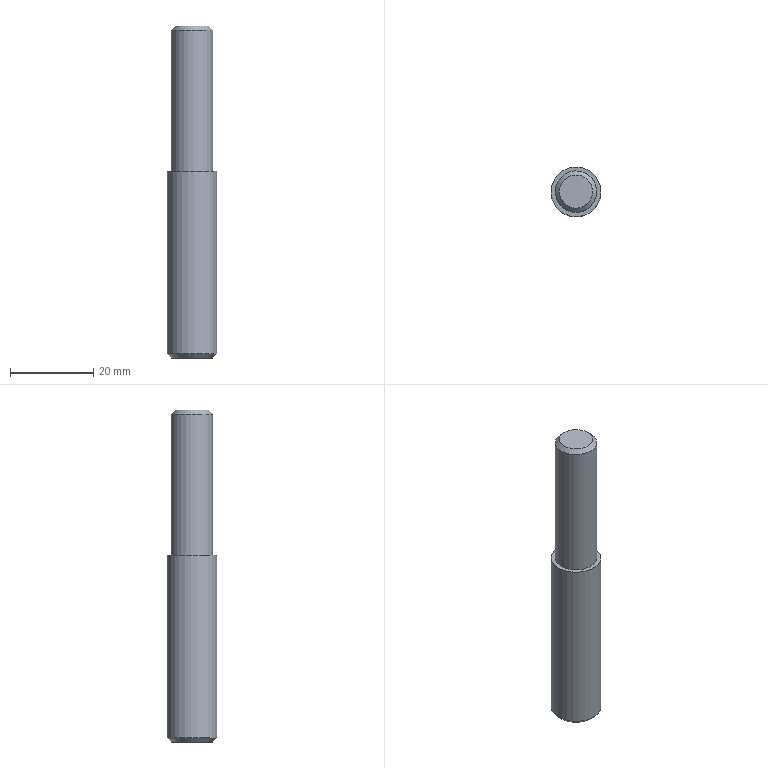Component | NX | PIN_FOR_TOGGLE_LEVER_2 | 1 solid | 7 faces | box 12 x 12 x 80 mm | volume 7806 mm3 | plane 3 | cylinder 2 | cone 2 | commonest cylinder face diameters 12 x1 10 x1
STEP:
#1=CARTESIAN_POINT('',(0.,0.,0.));
#2=DIRECTION('',(0.,0.,1.));
#3=DIRECTION('',(1.,0.,0.));
#4=AXIS2_PLACEMENT_3D('',#1,#2,#3);
#5=CARTESIAN_POINT('',(-2.434,171.826,43.728));
#6=VERTEX_POINT('',#5);
#7=CARTESIAN_POINT('',(0.,175.,43.728));
#8=DIRECTION('',(0.,0.,1.));
#9=DIRECTION('',(-0.6084,-0.7936,0.));
#10=AXIS2_PLACEMENT_3D('',#7,#8,#9);
#11=CIRCLE('',#10,4.);
#12=CARTESIAN_POINT('',(3.968,171.958,43.728));
#13=DIRECTION('',(0.,0.,1.));
#14=DIRECTION('',(-0.6084,-0.7936,0.));
#15=AXIS2_PLACEMENT_3D('',#12,#13,#14);
#16=PLANE('',#15);
#17=CARTESIAN_POINT('',(-0.,-5.));
#18=DIRECTION('',(1.,-0.));
#19=AXIS2_PLACEMENT_2D('',#17,#18);
#20=CIRCLE('',#19,4.);
#21=(GEOMETRIC_REPRESENTATION_CONTEXT(2)PARAMETRIC_REPRESENTATION_CONTEXT()REPRESENTATION_CONTEXT('',''));
#22=DEFINITIONAL_REPRESENTATION('',(#20),#21);
#23=PCURVE('',#16,#22);
#24=CARTESIAN_POINT('',(0.,175.,42.728));
#25=DIRECTION('',(0.,0.,-1.));
#26=DIRECTION('',(0.6084,0.7936,0.));
#27=AXIS2_PLACEMENT_3D('',#24,#25,#26);
#28=CONICAL_SURFACE('',#27,5.,0.7854);
#29=CARTESIAN_POINT('',(9.425,-1.));
#30=DIRECTION('',(-1.,0.));
#31=VECTOR('',#30,1.);
#32=LINE('',#29,#31);
#33=(GEOMETRIC_REPRESENTATION_CONTEXT(2)PARAMETRIC_REPRESENTATION_CONTEXT()REPRESENTATION_CONTEXT('',''));
#34=DEFINITIONAL_REPRESENTATION('',(#32),#33);
#35=PCURVE('',#28,#34);
#36=SURFACE_CURVE('',#11,(#23,#35),.PCURVE_S1.);
#37=EDGE_CURVE('',#6,#6,#36,.T.);
#38=ORIENTED_EDGE('',*,*,#37,.T.);
#39=EDGE_LOOP('',(#38));
#40=FACE_BOUND('',#39,.T.);
#41=ADVANCED_FACE('',(#40),#16,.T.);
#42=CARTESIAN_POINT('',(3.042,178.968,-36.272));
#43=VERTEX_POINT('',#42);
#44=CARTESIAN_POINT('',(0.,175.,-36.272));
#45=DIRECTION('',(0.,0.,-1.));
#46=DIRECTION('',(0.6084,0.7936,0.));
#47=AXIS2_PLACEMENT_3D('',#44,#45,#46);
#48=CIRCLE('',#47,5.);
#49=CARTESIAN_POINT('',(0.,175.,-36.272));
#50=DIRECTION('',(0.,0.,-1.));
#51=DIRECTION('',(0.6084,0.7936,0.));
#52=AXIS2_PLACEMENT_3D('',#49,#50,#51);
#53=PLANE('',#52);
#54=CARTESIAN_POINT('',(0.,0.));
#55=DIRECTION('',(1.,-0.));
#56=AXIS2_PLACEMENT_2D('',#54,#55);
#57=CIRCLE('',#56,5.);
#58=(GEOMETRIC_REPRESENTATION_CONTEXT(2)PARAMETRIC_REPRESENTATION_CONTEXT()REPRESENTATION_CONTEXT('',''));
#59=DEFINITIONAL_REPRESENTATION('',(#57),#58);
#60=PCURVE('',#53,#59);
#61=CARTESIAN_POINT('',(0.,175.,-36.272));
#62=DIRECTION('',(0.,0.,1.));
#63=DIRECTION('',(-0.6084,-0.7936,0.));
#64=AXIS2_PLACEMENT_3D('',#61,#62,#63);
#65=CONICAL_SURFACE('',#64,5.,0.7854);
#66=CARTESIAN_POINT('',(9.425,-0.));
#67=DIRECTION('',(-1.,0.));
#68=VECTOR('',#67,1.);
#69=LINE('',#66,#68);
#70=(GEOMETRIC_REPRESENTATION_CONTEXT(2)PARAMETRIC_REPRESENTATION_CONTEXT()REPRESENTATION_CONTEXT('',''));
#71=DEFINITIONAL_REPRESENTATION('',(#69),#70);
#72=PCURVE('',#65,#71);
#73=SURFACE_CURVE('',#48,(#60,#72),.PCURVE_S1.);
#74=EDGE_CURVE('',#43,#43,#73,.T.);
#75=ORIENTED_EDGE('',*,*,#74,.T.);
#76=EDGE_LOOP('',(#75));
#77=FACE_BOUND('',#76,.T.);
#78=ADVANCED_FACE('',(#77),#53,.T.);
#79=CARTESIAN_POINT('',(3.651,179.762,-35.272));
#80=VERTEX_POINT('',#79);
#81=CARTESIAN_POINT('',(0.,175.,-35.272));
#82=DIRECTION('',(0.,0.,1.));
#83=DIRECTION('',(0.6084,0.7936,0.));
#84=AXIS2_PLACEMENT_3D('',#81,#82,#83);
#85=CIRCLE('',#84,6.);
#86=CARTESIAN_POINT('',(0.,175.,-36.272));
#87=DIRECTION('',(0.,0.,-1.));
#88=DIRECTION('',(0.6084,0.7936,0.));
#89=AXIS2_PLACEMENT_3D('',#86,#87,#88);
#90=CYLINDRICAL_SURFACE('',#89,6.);
#91=CARTESIAN_POINT('',(6.283,-1.));
#92=DIRECTION('',(-1.,0.));
#93=VECTOR('',#92,1.);
#94=LINE('',#91,#93);
#95=(GEOMETRIC_REPRESENTATION_CONTEXT(2)PARAMETRIC_REPRESENTATION_CONTEXT()REPRESENTATION_CONTEXT('',''));
#96=DEFINITIONAL_REPRESENTATION('',(#94),#95);
#97=PCURVE('',#90,#96);
#98=CARTESIAN_POINT('',(3.142,1.));
#99=DIRECTION('',(1.,0.));
#100=VECTOR('',#99,1.);
#101=LINE('',#98,#100);
#102=(GEOMETRIC_REPRESENTATION_CONTEXT(2)PARAMETRIC_REPRESENTATION_CONTEXT()REPRESENTATION_CONTEXT('',''));
#103=DEFINITIONAL_REPRESENTATION('',(#101),#102);
#104=PCURVE('',#65,#103);
#105=SURFACE_CURVE('',#85,(#97,#104),.PCURVE_S1.);
#106=EDGE_CURVE('',#80,#80,#105,.T.);
#107=ORIENTED_EDGE('',*,*,#106,.T.);
#108=CARTESIAN_POINT('',(3.651,179.762,8.728));
#109=VERTEX_POINT('',#108);
#110=CARTESIAN_POINT('',(3.651,179.762,8.728));
#111=CARTESIAN_POINT('',(3.651,179.762,-35.272));
#112=B_SPLINE_CURVE_WITH_KNOTS('',1,(#110,#111),.UNSPECIFIED.,.F.,.F.,(2,2),(-45.,-1.),.PIECEWISE_BEZIER_KNOTS.);
#113=CARTESIAN_POINT('',(0.,0.));
#114=DIRECTION('',(0.,1.));
#115=VECTOR('',#114,1.);
#116=LINE('',#113,#115);
#117=(GEOMETRIC_REPRESENTATION_CONTEXT(2)PARAMETRIC_REPRESENTATION_CONTEXT()REPRESENTATION_CONTEXT('',''));
#118=DEFINITIONAL_REPRESENTATION('',(#116),#117);
#119=PCURVE('',#90,#118);
#120=CARTESIAN_POINT('',(6.283,0.));
#121=DIRECTION('',(0.,1.));
#122=VECTOR('',#121,1.);
#123=LINE('',#120,#122);
#124=(GEOMETRIC_REPRESENTATION_CONTEXT(2)PARAMETRIC_REPRESENTATION_CONTEXT()REPRESENTATION_CONTEXT('',''));
#125=DEFINITIONAL_REPRESENTATION('',(#123),#124);
#126=PCURVE('',#90,#125);
#127=SEAM_CURVE('',#112,(#119,#126),.PCURVE_S1.);
#128=EDGE_CURVE('',#109,#80,#127,.T.);
#129=ORIENTED_EDGE('',*,*,#128,.F.);
#130=CARTESIAN_POINT('',(0.,175.,8.728));
#131=DIRECTION('',(0.,0.,-1.));
#132=DIRECTION('',(0.6084,0.7936,0.));
#133=AXIS2_PLACEMENT_3D('',#130,#131,#132);
#134=CIRCLE('',#133,6.);
#135=CARTESIAN_POINT('',(0.,-45.));
#136=DIRECTION('',(1.,0.));
#137=VECTOR('',#136,1.);
#138=LINE('',#135,#137);
#139=(GEOMETRIC_REPRESENTATION_CONTEXT(2)PARAMETRIC_REPRESENTATION_CONTEXT()REPRESENTATION_CONTEXT('',''));
#140=DEFINITIONAL_REPRESENTATION('',(#138),#139);
#141=PCURVE('',#90,#140);
#142=CARTESIAN_POINT('',(4.762,171.349,8.728));
#143=DIRECTION('',(0.,0.,1.));
#144=DIRECTION('',(-0.6084,-0.7936,0.));
#145=AXIS2_PLACEMENT_3D('',#142,#143,#144);
#146=PLANE('',#145);
#147=CARTESIAN_POINT('',(-6.,-6.));
#148=CARTESIAN_POINT('',(-6.,4.392));
#149=CARTESIAN_POINT('',(3.,-0.8038));
#150=CARTESIAN_POINT('',(12.,-6.));
#151=CARTESIAN_POINT('',(3.,-11.196));
#152=CARTESIAN_POINT('',(-6.,-16.392));
#153=CARTESIAN_POINT('',(-6.,-6.));
#154=(BOUNDED_CURVE()B_SPLINE_CURVE(2,(#147,#148,#149,#150,#151,#152,#153),.UNSPECIFIED.,.T.,.F.)B_SPLINE_CURVE_WITH_KNOTS((1,2,2,2,2,1),(-2.094,0.,2.094,4.189,6.283,8.378),.UNSPECIFIED.)CURVE()GEOMETRIC_REPRESENTATION_ITEM()RATIONAL_B_SPLINE_CURVE((1.,0.5,1.,0.5,1.,0.5,1.))REPRESENTATION_ITEM(''));
#155=(GEOMETRIC_REPRESENTATION_CONTEXT(2)PARAMETRIC_REPRESENTATION_CONTEXT()REPRESENTATION_CONTEXT('',''));
#156=DEFINITIONAL_REPRESENTATION('',(#154),#155);
#157=PCURVE('',#146,#156);
#158=SURFACE_CURVE('',#134,(#141,#157),.PCURVE_S1.);
#159=EDGE_CURVE('',#109,#109,#158,.T.);
#160=ORIENTED_EDGE('',*,*,#159,.T.);
#161=ORIENTED_EDGE('',*,*,#128,.T.);
#162=EDGE_LOOP('',(#107,#129,#160,#161));
#163=FACE_BOUND('',#162,.T.);
#164=ADVANCED_FACE('',(#163),#90,.T.);
#165=CARTESIAN_POINT('',(3.042,178.968,8.728));
#166=VERTEX_POINT('',#165);
#167=CARTESIAN_POINT('',(0.,175.,8.728));
#168=DIRECTION('',(0.,0.,-1.));
#169=DIRECTION('',(0.6084,0.7936,0.));
#170=AXIS2_PLACEMENT_3D('',#167,#168,#169);
#171=CIRCLE('',#170,5.);
#172=CARTESIAN_POINT('',(-5.,-6.));
#173=CARTESIAN_POINT('',(-5.,2.66));
#174=CARTESIAN_POINT('',(2.5,-1.67));
#175=CARTESIAN_POINT('',(10.,-6.));
#176=CARTESIAN_POINT('',(2.5,-10.33));
#177=CARTESIAN_POINT('',(-5.,-14.66));
#178=CARTESIAN_POINT('',(-5.,-6.));
#179=(BOUNDED_CURVE()B_SPLINE_CURVE(2,(#172,#173,#174,#175,#176,#177,#178),.UNSPECIFIED.,.T.,.F.)B_SPLINE_CURVE_WITH_KNOTS((1,2,2,2,2,1),(-2.094,0.,2.094,4.189,6.283,8.378),.UNSPECIFIED.)CURVE()GEOMETRIC_REPRESENTATION_ITEM()RATIONAL_B_SPLINE_CURVE((1.,0.5,1.,0.5,1.,0.5,1.))REPRESENTATION_ITEM(''));
#180=(GEOMETRIC_REPRESENTATION_CONTEXT(2)PARAMETRIC_REPRESENTATION_CONTEXT()REPRESENTATION_CONTEXT('',''));
#181=DEFINITIONAL_REPRESENTATION('',(#179),#180);
#182=PCURVE('',#146,#181);
#183=CARTESIAN_POINT('',(0.,175.,-36.272));
#184=DIRECTION('',(0.,0.,-1.));
#185=DIRECTION('',(0.6084,0.7936,0.));
#186=AXIS2_PLACEMENT_3D('',#183,#184,#185);
#187=CYLINDRICAL_SURFACE('',#186,5.);
#188=CARTESIAN_POINT('',(0.,-45.));
#189=DIRECTION('',(1.,0.));
#190=VECTOR('',#189,1.);
#191=LINE('',#188,#190);
#192=(GEOMETRIC_REPRESENTATION_CONTEXT(2)PARAMETRIC_REPRESENTATION_CONTEXT()REPRESENTATION_CONTEXT('',''));
#193=DEFINITIONAL_REPRESENTATION('',(#191),#192);
#194=PCURVE('',#187,#193);
#195=SURFACE_CURVE('',#171,(#182,#194),.PCURVE_S1.);
#196=EDGE_CURVE('',#166,#166,#195,.T.);
#197=ORIENTED_EDGE('',*,*,#196,.T.);
#198=EDGE_LOOP('',(#197));
#199=FACE_BOUND('',#198,.T.);
#200=ORIENTED_EDGE('',*,*,#159,.F.);
#201=EDGE_LOOP('',(#200));
#202=FACE_BOUND('',#201,.T.);
#203=ADVANCED_FACE('',(#199,#202),#146,.T.);
#204=CARTESIAN_POINT('',(-3.042,171.032,42.728));
#205=VERTEX_POINT('',#204);
#206=CARTESIAN_POINT('',(3.042,178.968,42.728));
#207=VERTEX_POINT('',#206);
#208=CARTESIAN_POINT('',(0.,175.,42.728));
#209=DIRECTION('',(0.,0.,-1.));
#210=DIRECTION('',(-0.6084,-0.7936,0.));
#211=AXIS2_PLACEMENT_3D('',#208,#209,#210);
#212=CIRCLE('',#211,5.);
#213=CARTESIAN_POINT('',(3.142,-79.));
#214=DIRECTION('',(1.,0.));
#215=VECTOR('',#214,1.);
#216=LINE('',#213,#215);
#217=(GEOMETRIC_REPRESENTATION_CONTEXT(2)PARAMETRIC_REPRESENTATION_CONTEXT()REPRESENTATION_CONTEXT('',''));
#218=DEFINITIONAL_REPRESENTATION('',(#216),#217);
#219=PCURVE('',#187,#218);
#220=CARTESIAN_POINT('',(3.142,0.));
#221=DIRECTION('',(1.,-0.));
#222=VECTOR('',#221,1.);
#223=LINE('',#220,#222);
#224=(GEOMETRIC_REPRESENTATION_CONTEXT(2)PARAMETRIC_REPRESENTATION_CONTEXT()REPRESENTATION_CONTEXT('',''));
#225=DEFINITIONAL_REPRESENTATION('',(#223),#224);
#226=PCURVE('',#28,#225);
#227=SURFACE_CURVE('',#212,(#219,#226),.PCURVE_S1.);
#228=EDGE_CURVE('',#205,#207,#227,.T.);
#229=ORIENTED_EDGE('',*,*,#228,.T.);
#230=CARTESIAN_POINT('',(3.042,178.968,42.728));
#231=CARTESIAN_POINT('',(3.042,178.968,8.728));
#232=B_SPLINE_CURVE_WITH_KNOTS('',1,(#230,#231),.UNSPECIFIED.,.F.,.F.,(2,2),(-79.,-45.),.PIECEWISE_BEZIER_KNOTS.);
#233=CARTESIAN_POINT('',(6.283,0.));
#234=DIRECTION('',(0.,1.));
#235=VECTOR('',#234,1.);
#236=LINE('',#233,#235);
#237=(GEOMETRIC_REPRESENTATION_CONTEXT(2)PARAMETRIC_REPRESENTATION_CONTEXT()REPRESENTATION_CONTEXT('',''));
#238=DEFINITIONAL_REPRESENTATION('',(#236),#237);
#239=PCURVE('',#187,#238);
#240=CARTESIAN_POINT('',(0.,0.));
#241=DIRECTION('',(0.,1.));
#242=VECTOR('',#241,1.);
#243=LINE('',#240,#242);
#244=(GEOMETRIC_REPRESENTATION_CONTEXT(2)PARAMETRIC_REPRESENTATION_CONTEXT()REPRESENTATION_CONTEXT('',''));
#245=DEFINITIONAL_REPRESENTATION('',(#243),#244);
#246=PCURVE('',#187,#245);
#247=SEAM_CURVE('',#232,(#239,#246),.PCURVE_S1.);
#248=EDGE_CURVE('',#207,#166,#247,.T.);
#249=ORIENTED_EDGE('',*,*,#248,.T.);
#250=ORIENTED_EDGE('',*,*,#196,.F.);
#251=ORIENTED_EDGE('',*,*,#248,.F.);
#252=CARTESIAN_POINT('',(0.,175.,42.728));
#253=DIRECTION('',(0.,0.,-1.));
#254=DIRECTION('',(-0.6084,-0.7936,0.));
#255=AXIS2_PLACEMENT_3D('',#252,#253,#254);
#256=CIRCLE('',#255,5.);
#257=CARTESIAN_POINT('',(-3.142,-79.));
#258=DIRECTION('',(1.,0.));
#259=VECTOR('',#258,1.);
#260=LINE('',#257,#259);
#261=(GEOMETRIC_REPRESENTATION_CONTEXT(2)PARAMETRIC_REPRESENTATION_CONTEXT()REPRESENTATION_CONTEXT('',''));
#262=DEFINITIONAL_REPRESENTATION('',(#260),#261);
#263=PCURVE('',#187,#262);
#264=CARTESIAN_POINT('',(3.142,-0.));
#265=DIRECTION('',(1.,0.));
#266=VECTOR('',#265,1.);
#267=LINE('',#264,#266);
#268=(GEOMETRIC_REPRESENTATION_CONTEXT(2)PARAMETRIC_REPRESENTATION_CONTEXT()REPRESENTATION_CONTEXT('',''));
#269=DEFINITIONAL_REPRESENTATION('',(#267),#268);
#270=PCURVE('',#28,#269);
#271=SURFACE_CURVE('',#256,(#263,#270),.PCURVE_S1.);
#272=EDGE_CURVE('',#207,#205,#271,.T.);
#273=ORIENTED_EDGE('',*,*,#272,.T.);
#274=EDGE_LOOP('',(#229,#249,#250,#251,#273));
#275=FACE_BOUND('',#274,.T.);
#276=ADVANCED_FACE('',(#275),#187,.T.);
#277=ORIENTED_EDGE('',*,*,#106,.F.);
#278=CARTESIAN_POINT('',(3.042,178.968,-36.272));
#279=CARTESIAN_POINT('',(3.651,179.762,-35.272));
#280=B_SPLINE_CURVE_WITH_KNOTS('',1,(#278,#279),.UNSPECIFIED.,.F.,.F.,(2,2),(-0.,1.414),.PIECEWISE_BEZIER_KNOTS.);
#281=CARTESIAN_POINT('',(3.142,0.));
#282=DIRECTION('',(0.,1.));
#283=VECTOR('',#282,1.);
#284=LINE('',#281,#283);
#285=(GEOMETRIC_REPRESENTATION_CONTEXT(2)PARAMETRIC_REPRESENTATION_CONTEXT()REPRESENTATION_CONTEXT('',''));
#286=DEFINITIONAL_REPRESENTATION('',(#284),#285);
#287=PCURVE('',#65,#286);
#288=CARTESIAN_POINT('',(9.425,0.));
#289=DIRECTION('',(0.,1.));
#290=VECTOR('',#289,1.);
#291=LINE('',#288,#290);
#292=(GEOMETRIC_REPRESENTATION_CONTEXT(2)PARAMETRIC_REPRESENTATION_CONTEXT()REPRESENTATION_CONTEXT('',''));
#293=DEFINITIONAL_REPRESENTATION('',(#291),#292);
#294=PCURVE('',#65,#293);
#295=SEAM_CURVE('',#280,(#287,#294),.PCURVE_S1.);
#296=EDGE_CURVE('',#43,#80,#295,.T.);
#297=ORIENTED_EDGE('',*,*,#296,.F.);
#298=ORIENTED_EDGE('',*,*,#74,.F.);
#299=ORIENTED_EDGE('',*,*,#296,.T.);
#300=EDGE_LOOP('',(#277,#297,#298,#299));
#301=FACE_BOUND('',#300,.T.);
#302=ADVANCED_FACE('',(#301),#65,.T.);
#303=ORIENTED_EDGE('',*,*,#37,.F.);
#304=CARTESIAN_POINT('',(-2.434,171.826,43.728));
#305=CARTESIAN_POINT('',(-3.042,171.032,42.728));
#306=B_SPLINE_CURVE_WITH_KNOTS('',1,(#304,#305),.UNSPECIFIED.,.F.,.F.,(2,2),(-1.414,0.),.PIECEWISE_BEZIER_KNOTS.);
#307=CARTESIAN_POINT('',(9.425,0.));
#308=DIRECTION('',(0.,1.));
#309=VECTOR('',#308,1.);
#310=LINE('',#307,#309);
#311=(GEOMETRIC_REPRESENTATION_CONTEXT(2)PARAMETRIC_REPRESENTATION_CONTEXT()REPRESENTATION_CONTEXT('',''));
#312=DEFINITIONAL_REPRESENTATION('',(#310),#311);
#313=PCURVE('',#28,#312);
#314=CARTESIAN_POINT('',(3.142,0.));
#315=DIRECTION('',(0.,1.));
#316=VECTOR('',#315,1.);
#317=LINE('',#314,#316);
#318=(GEOMETRIC_REPRESENTATION_CONTEXT(2)PARAMETRIC_REPRESENTATION_CONTEXT()REPRESENTATION_CONTEXT('',''));
#319=DEFINITIONAL_REPRESENTATION('',(#317),#318);
#320=PCURVE('',#28,#319);
#321=SEAM_CURVE('',#306,(#313,#320),.PCURVE_S1.);
#322=EDGE_CURVE('',#6,#205,#321,.T.);
#323=ORIENTED_EDGE('',*,*,#322,.T.);
#324=ORIENTED_EDGE('',*,*,#272,.F.);
#325=ORIENTED_EDGE('',*,*,#228,.F.);
#326=ORIENTED_EDGE('',*,*,#322,.F.);
#327=EDGE_LOOP('',(#303,#323,#324,#325,#326));
#328=FACE_BOUND('',#327,.T.);
#329=ADVANCED_FACE('',(#328),#28,.T.);
#330=CLOSED_SHELL('',(#41,#78,#164,#203,#276,#302,#329));
#331=MANIFOLD_SOLID_BREP('',#330);
#332=(LENGTH_UNIT()NAMED_UNIT(*)SI_UNIT(.MILLI.,.METRE.));
#333=UNCERTAINTY_MEASURE_WITH_UNIT(LENGTH_MEASURE(0.00001),#332,'','');
#334=(NAMED_UNIT(*)PLANE_ANGLE_UNIT()SI_UNIT($,.RADIAN.));
#335=(NAMED_UNIT(*)SI_UNIT($,.STERADIAN.)SOLID_ANGLE_UNIT());
#336=(GEOMETRIC_REPRESENTATION_CONTEXT(3)GLOBAL_UNCERTAINTY_ASSIGNED_CONTEXT((#333))GLOBAL_UNIT_ASSIGNED_CONTEXT((#332,#334,#335))REPRESENTATION_CONTEXT('',''));
#337=ADVANCED_BREP_SHAPE_REPRESENTATION('',(#4,#331),#336);